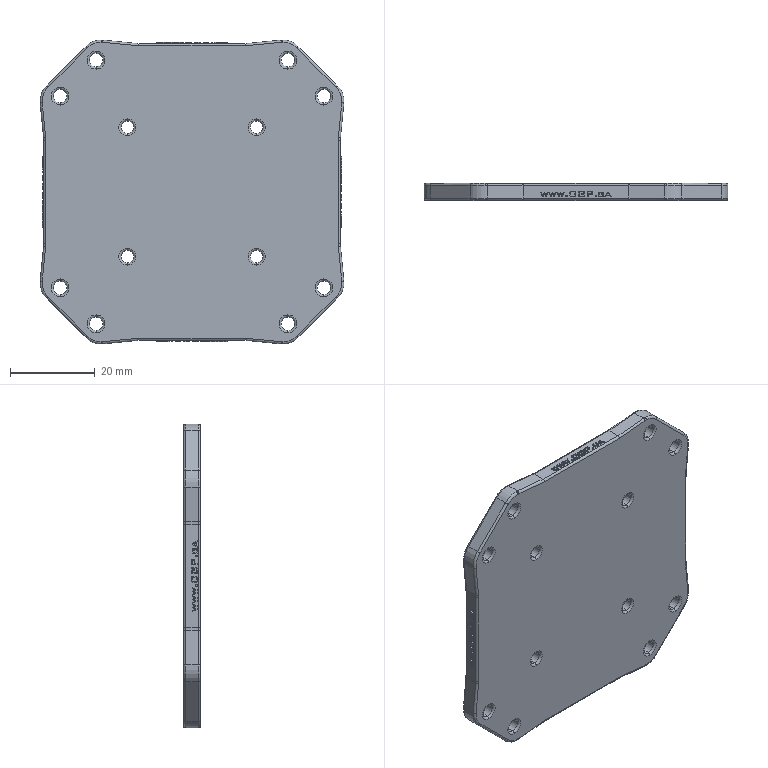Component | SolidWorks | 1.Spider base-2 | 1 solid | 908 faces | box 71.71 x 4 x 71.71 mm | volume 10782 mm3 | plane 532 | cylinder 136 | torus 128 | spline 112 | commonest cylinder face diameters 1 x72 6 x20 10 x20 3.2 x16 3 x8